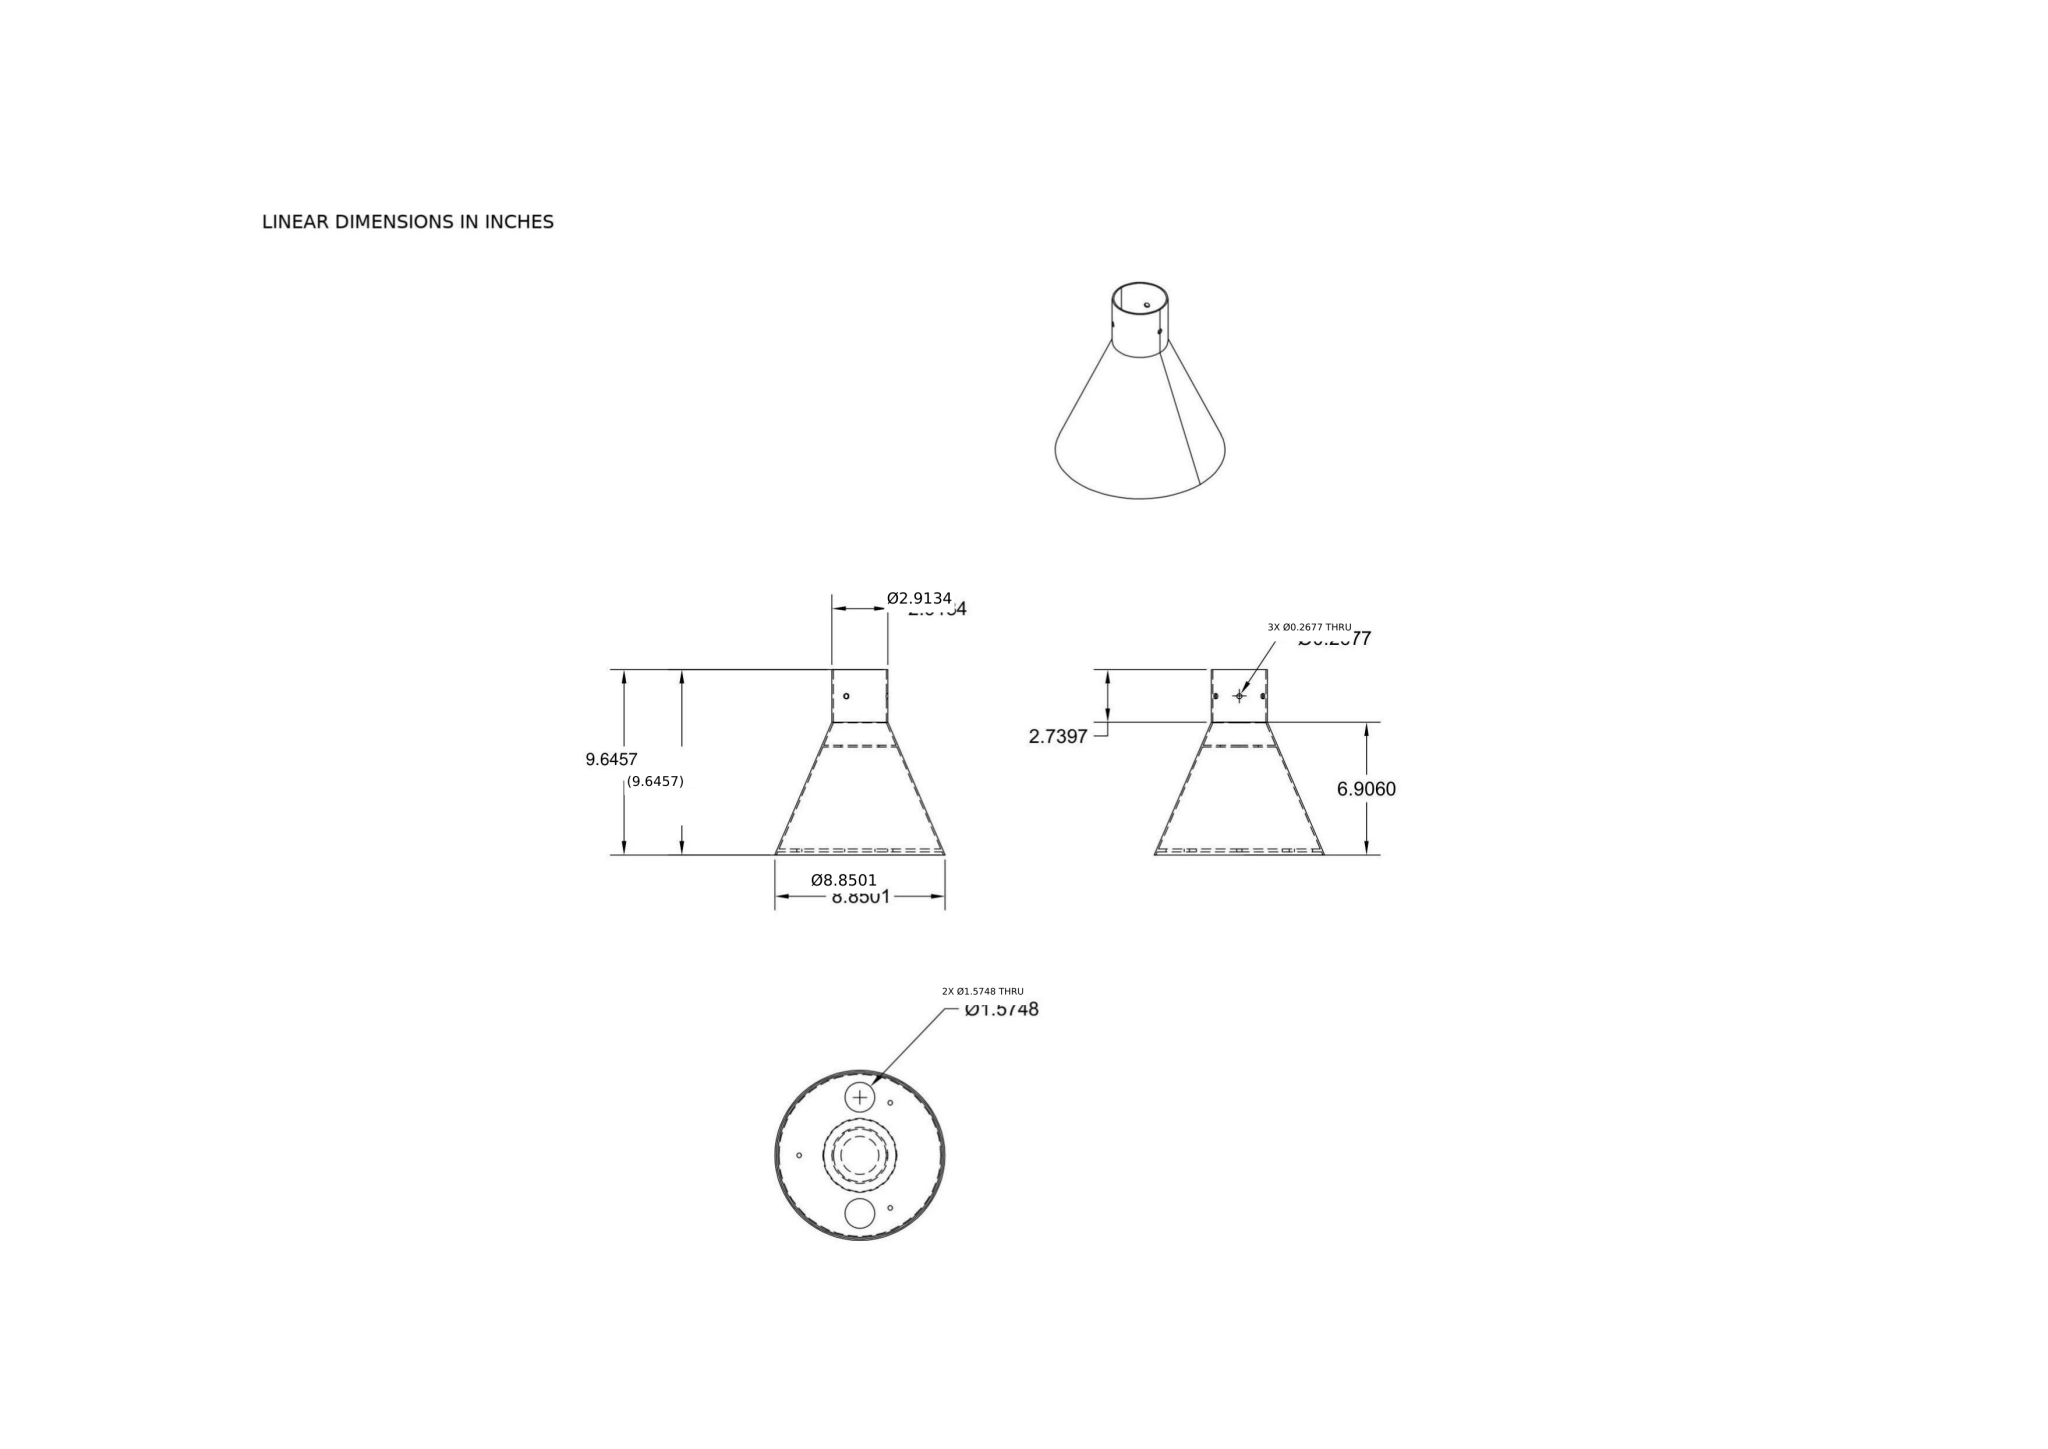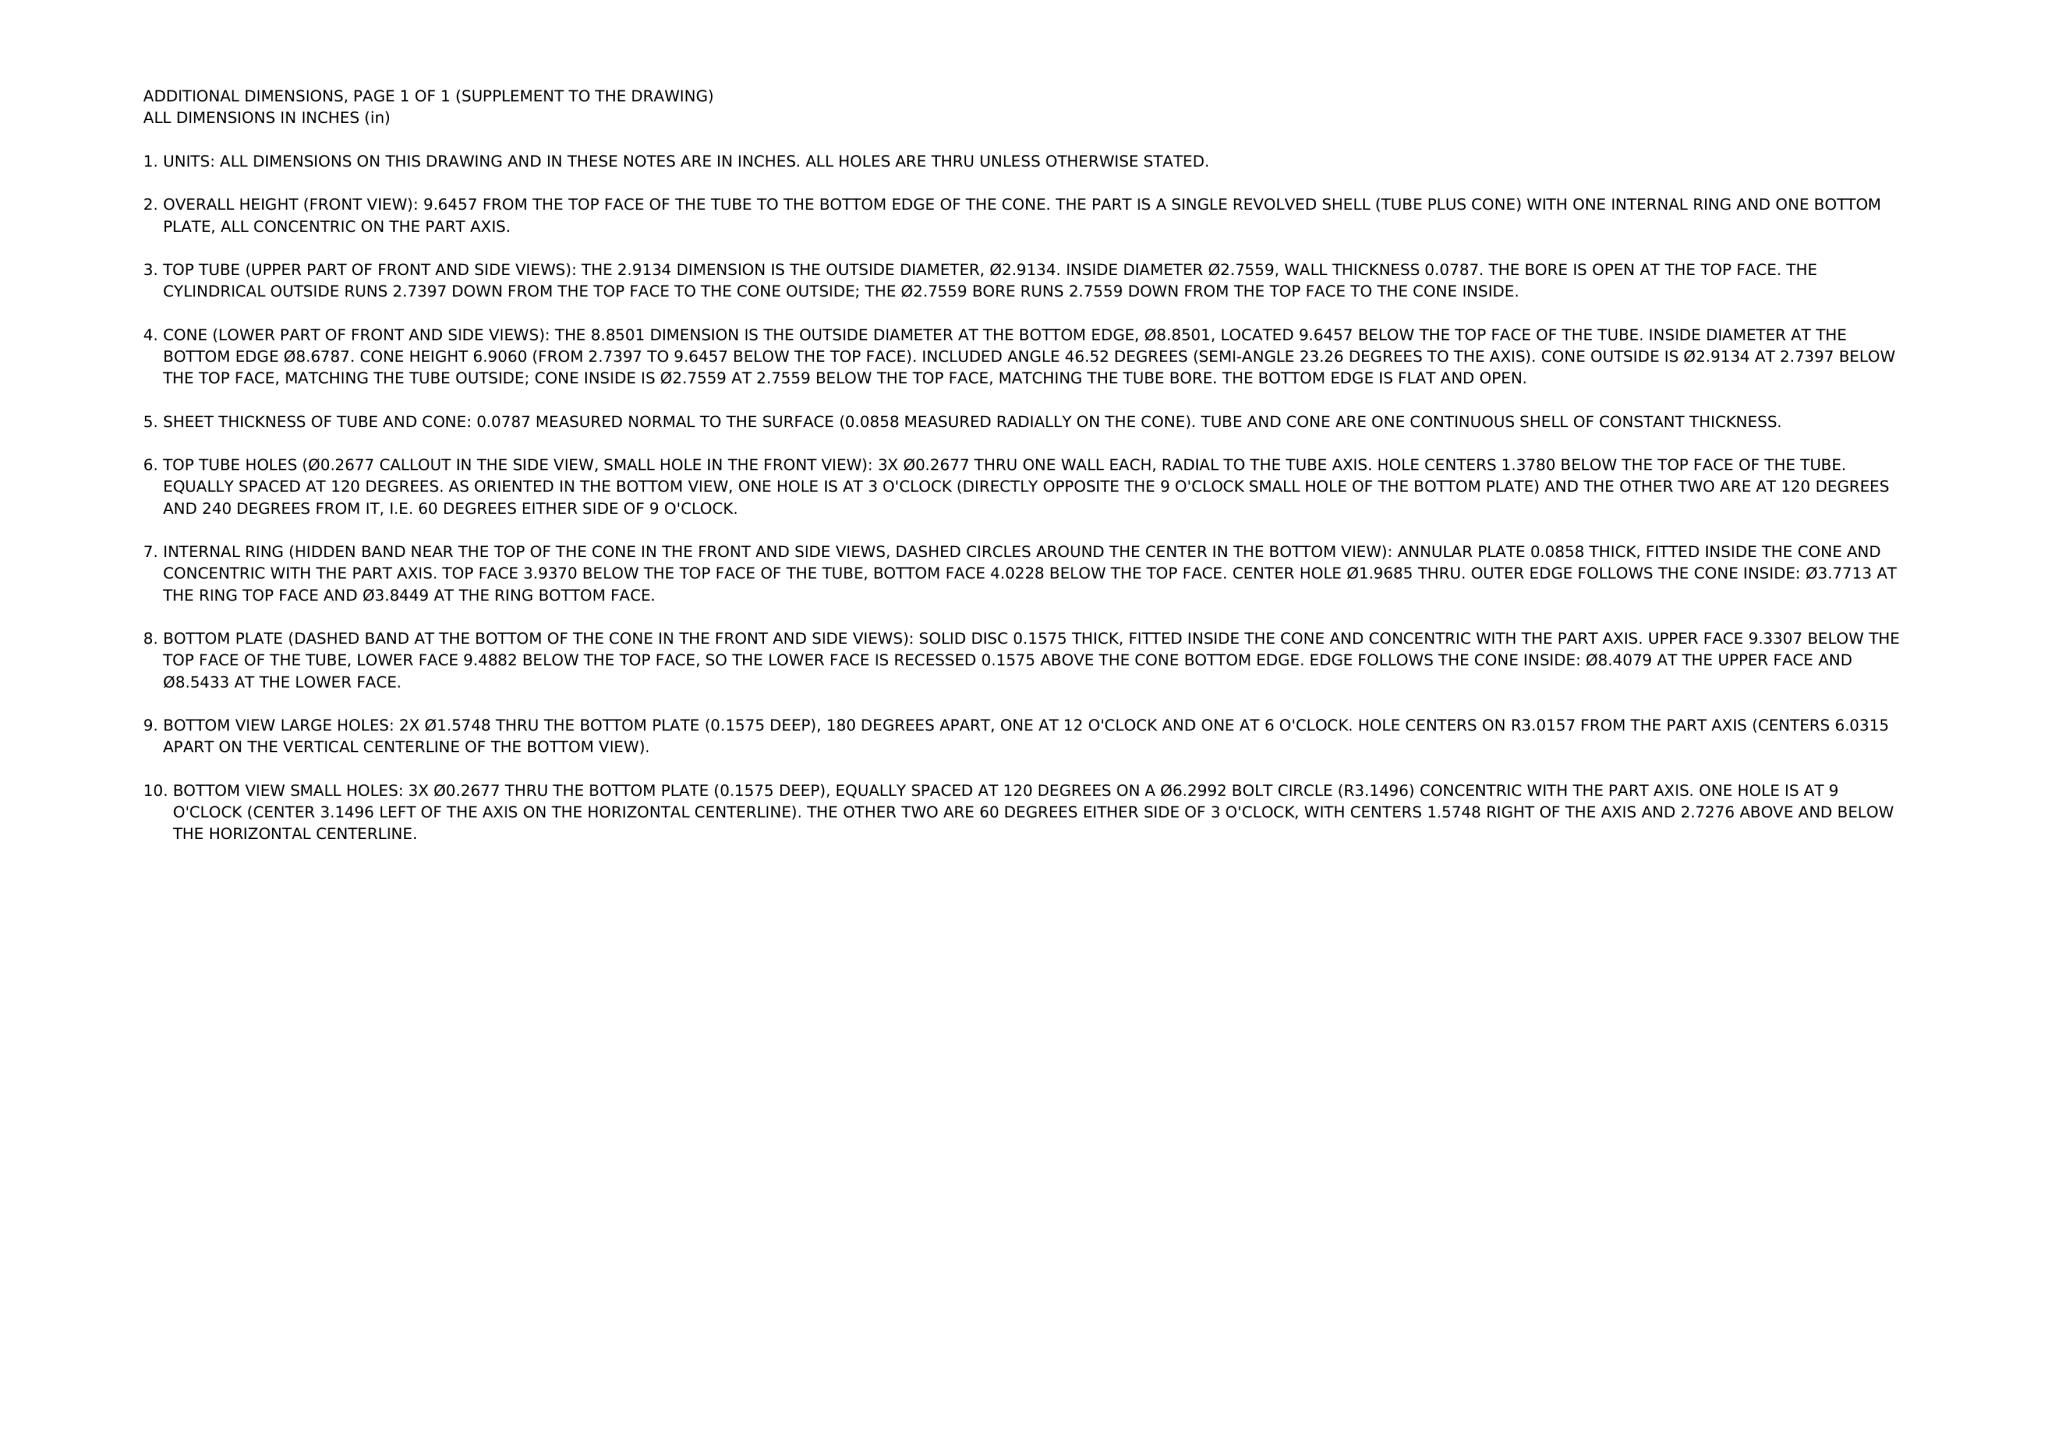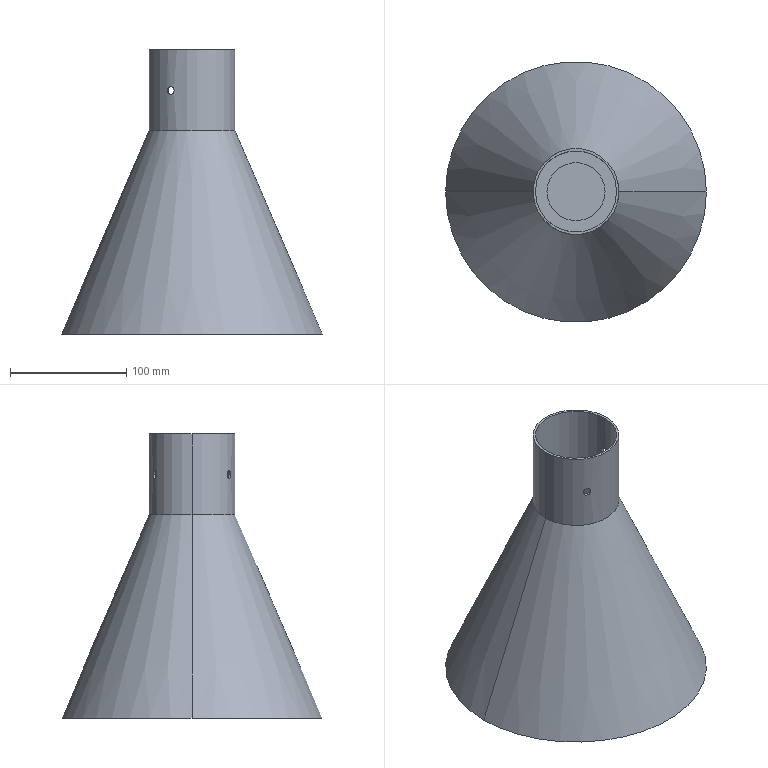Part | NX | mm | 1 solid | 36 faces | box 224.79 x 224.79 x 245 mm | volume 354701 mm3 | cylinder 22 | cone 8 | plane 6 | commonest cylinder face diameters 6.8 x12 40 x4 74 x2 70 x2 50 x2